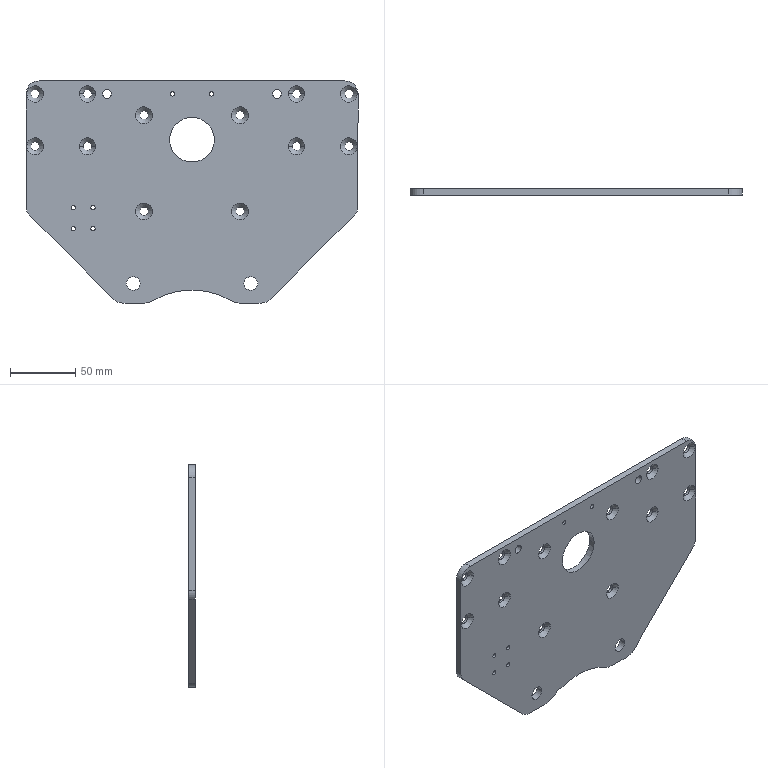Component | SolidWorks | QX1-03-BJMotorMountingPlate-1 | 1 solid | 88 faces | volume 179177 mm3 | cylinder 55 | cone 24 | plane 9 | commonest cylinder face diameters 6.6 x28 3.3 x12 20 x8 10.5 x4 34.3 x2 120 x1 | material 201 Annealed Stainless Steel (SS)